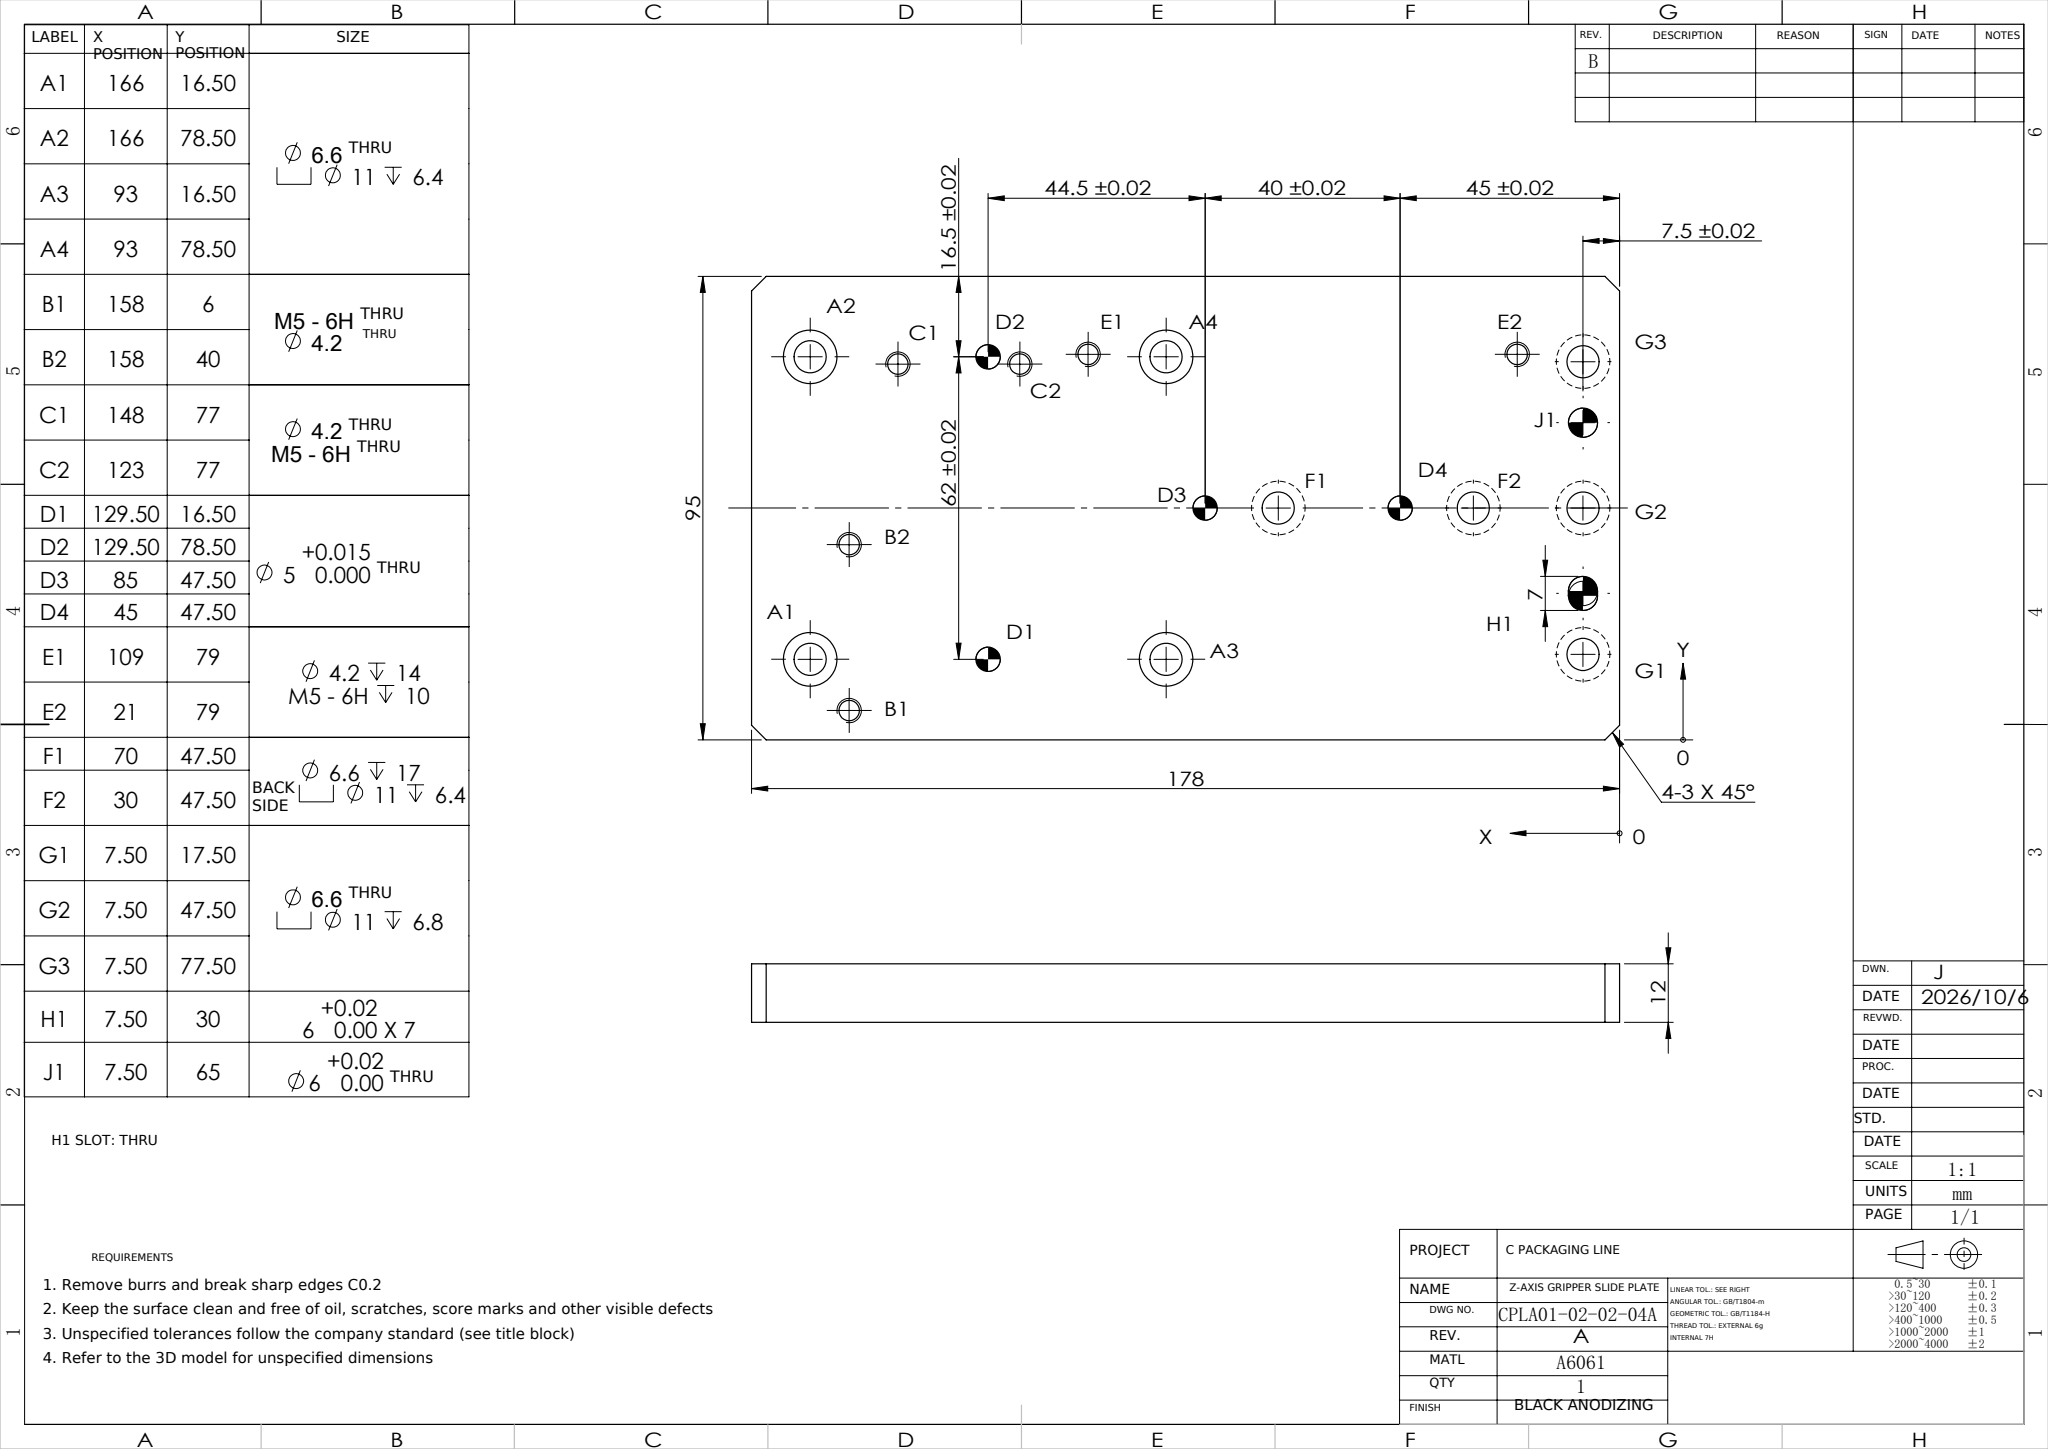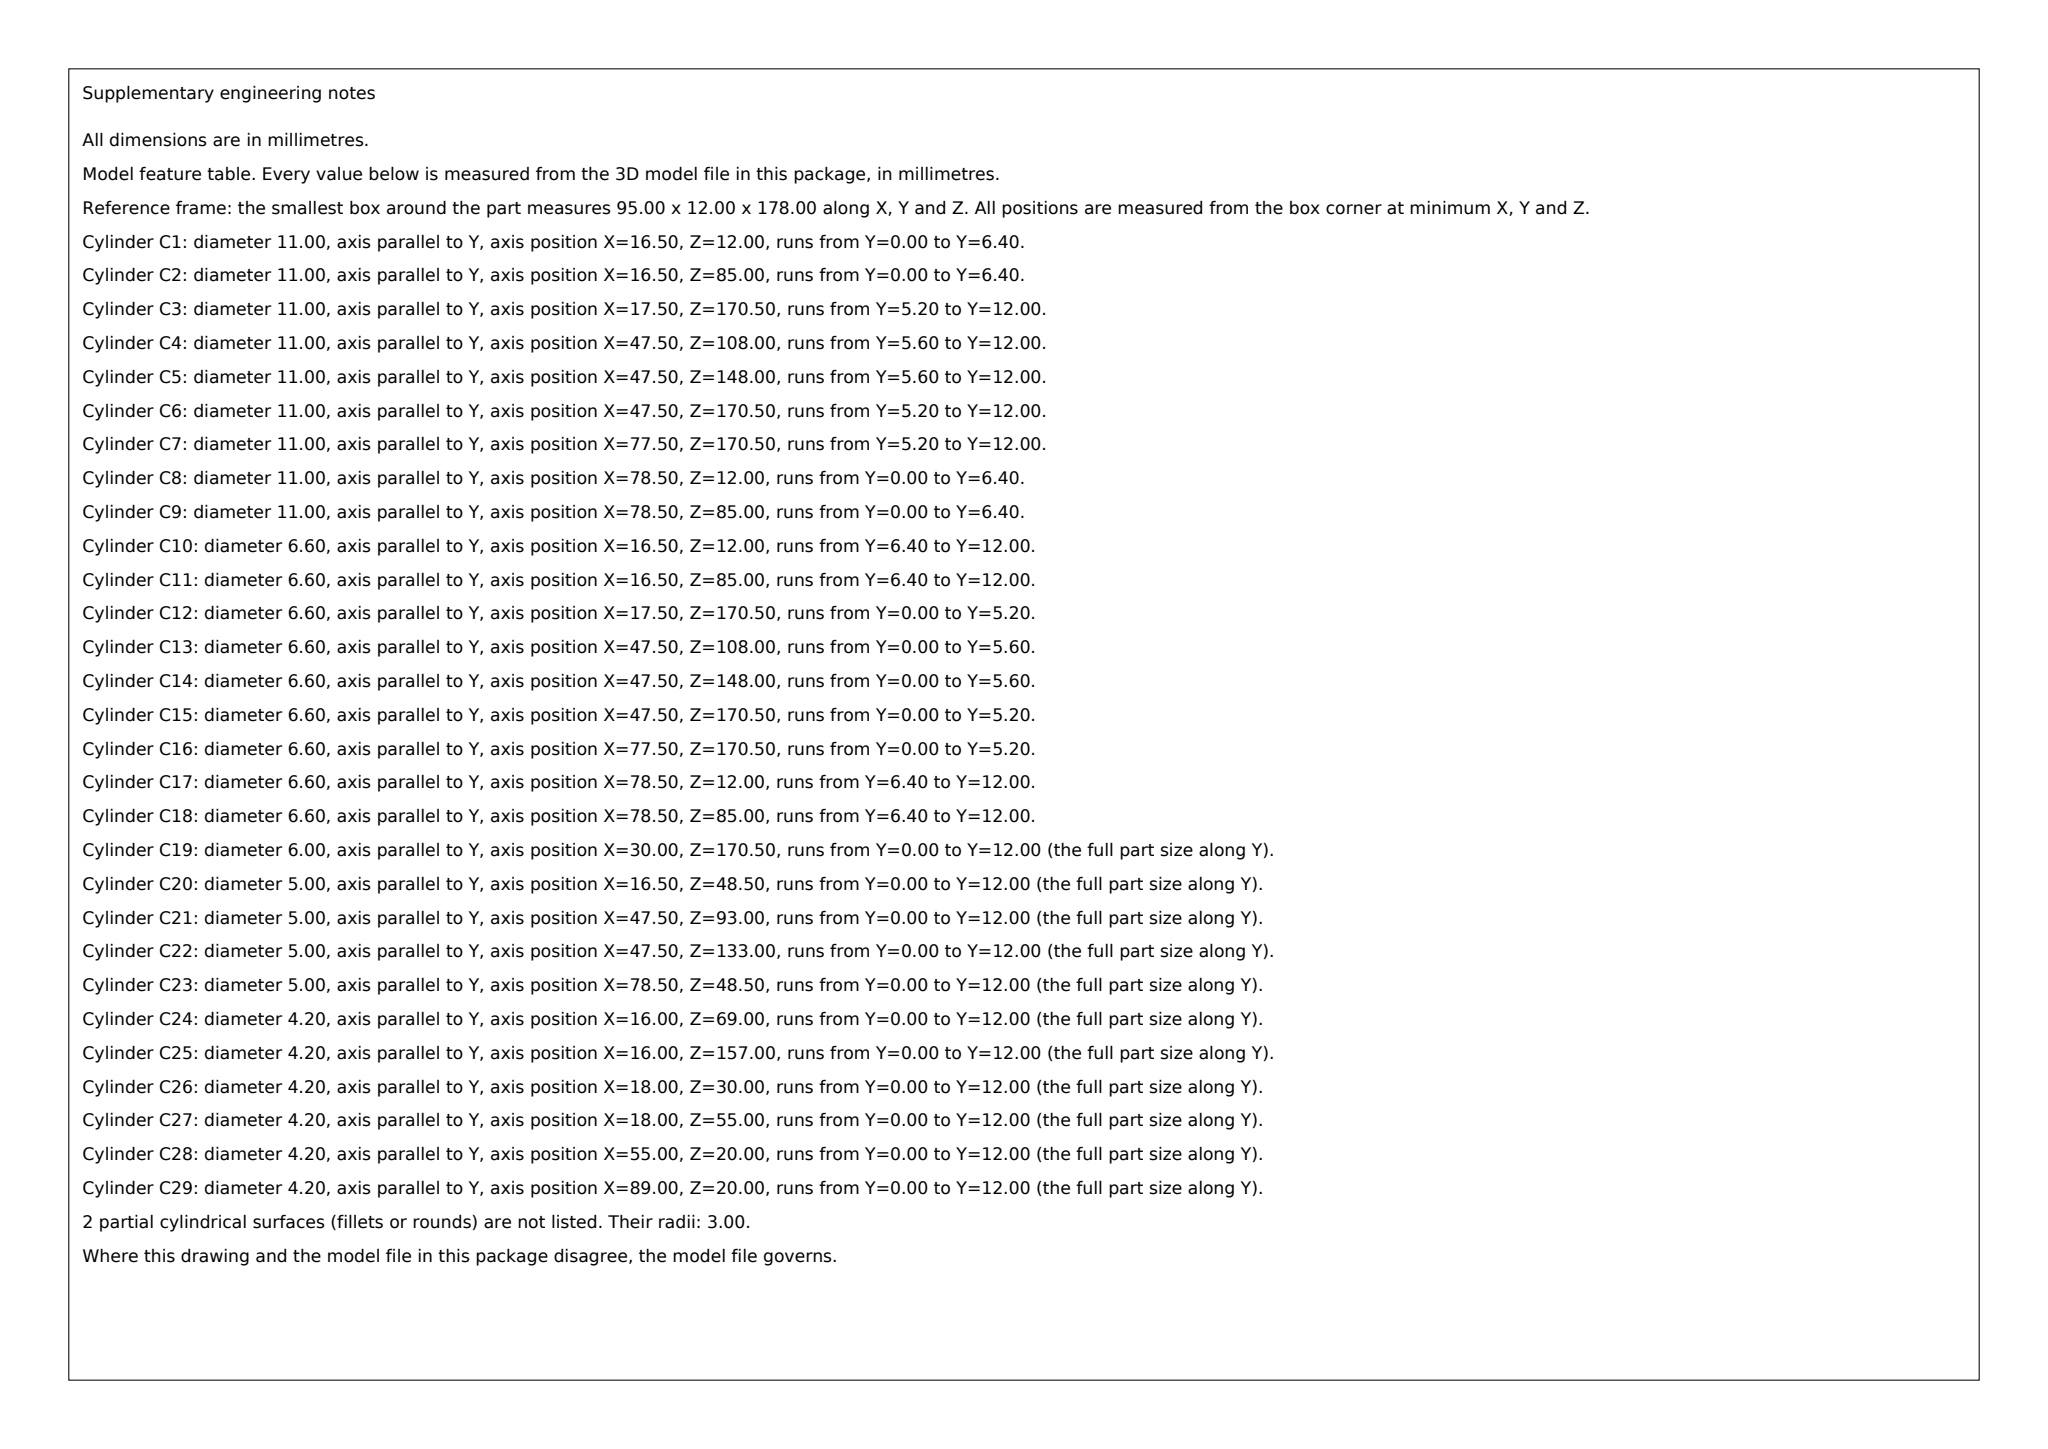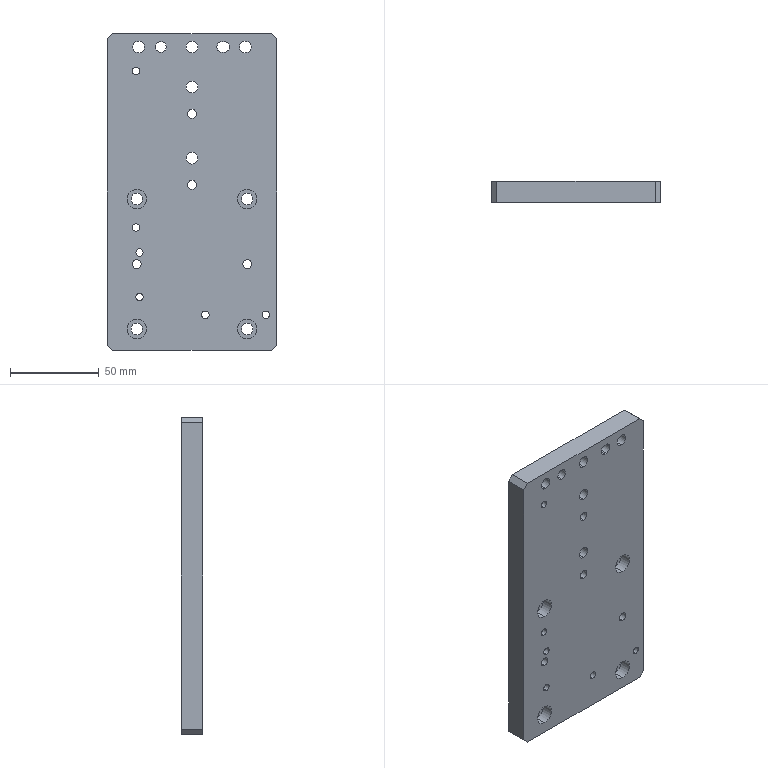Part | SolidWorks | mm | 1 solid | 81 faces | box 95 x 12 x 178 mm | volume 192742 mm3 | cylinder 60 | plane 21 | commonest cylinder face diameters 11 x18 6.6 x18 4.2 x12 5 x8 6 x4
build123d program:
from build123d import *

# Parameters (mm, degrees)
SKETCH1_W                                         = 95
SKETCH1_H                                         = 178
BOSS_EXTRUDE1_DEPTH                               = 12
M6_HEX_SOCKET_HEAD_CAP_SCREW_CBORE2_D             = 6.6
M6_HEX_SOCKET_HEAD_CAP_SCREW_CBORE2_CBORE_D       = 11
M6_HEX_SOCKET_HEAD_CAP_SCREW_CBORE2_CBORE_DEPTH   = 6.4
M6_HEX_SOCKET_HEAD_CAP_SCREW_CBORE1_D             = 6.6
M6_HEX_SOCKET_HEAD_CAP_SCREW_CBORE1_DEPTH         = 17
M6_HEX_SOCKET_HEAD_CAP_SCREW_CBORE1_CBORE_D       = 11
M6_HEX_SOCKET_HEAD_CAP_SCREW_CBORE1_CBORE_DEPTH   = 6.4
M6_HEX_SOCKET_HEAD_CAP_SCREW_CBORE1_TIP           = 1.983
M5_TAPPED_HOLE1_D                                 = 4.2
M5_TAPPED_HOLE1_DEPTH                             = 14
M5_TAPPED_HOLE1_TIP                               = 1.262
CHAMFER1_SIZE                                     = 3
M5_TAPPED_HOLE3_D                                 = 4.2
M5_TAPPED_HOLE4_D                                 = 4.2
F_5_0MM_DOWEL_PIN_HOLE1_D                         = 5
F_5_0MM_DOWEL_PIN_HOLE3_D                         = 5
M6_HEX_SOCKET_HEAD_CAP_SCREW_CBORE1_2_D           = 6.6
M6_HEX_SOCKET_HEAD_CAP_SCREW_CBORE1_2_CBORE_D     = 11
M6_HEX_SOCKET_HEAD_CAP_SCREW_CBORE1_2_CBORE_DEPTH = 6.8
SKETCH24_R                                        = 3
CUT_EXTRUDE1_DEPTH                                = 102.594


with BuildPart() as part:
    # Sketch1 → Boss-Extrude1 (new body)
    with BuildSketch(Plane(origin=(0, 0, 0), x_dir=(1, 0, 0), z_dir=(0, 1, 0))):
        Rectangle(SKETCH1_W, SKETCH1_H)
    extrude(amount=BOSS_EXTRUDE1_DEPTH)

    # M6 Hex Socket Head Cap Screw CBORE2 (through all)
    with Locations(Plane(origin=(0, 0, 0), x_dir=(-1, 0, 0), z_dir=(0, -1, 0))):
        with Locations((-31, 77), (-31, 4), (31, 77), (31, 4)):
            CounterBoreHole(M6_HEX_SOCKET_HEAD_CAP_SCREW_CBORE2_D / 2, M6_HEX_SOCKET_HEAD_CAP_SCREW_CBORE2_CBORE_D / 2, M6_HEX_SOCKET_HEAD_CAP_SCREW_CBORE2_CBORE_DEPTH)

    # M6 Hex Socket Head Cap Screw CBORE1
    with Locations(Plane(origin=(0, 12, 0), x_dir=(1, 0, 0), z_dir=(0, 1, 0))):
        with Locations((0, -59), (0, -19)):
            CounterBoreHole(M6_HEX_SOCKET_HEAD_CAP_SCREW_CBORE1_D / 2, M6_HEX_SOCKET_HEAD_CAP_SCREW_CBORE1_CBORE_D / 2, M6_HEX_SOCKET_HEAD_CAP_SCREW_CBORE1_CBORE_DEPTH, depth=M6_HEX_SOCKET_HEAD_CAP_SCREW_CBORE1_DEPTH)
            with Locations((0, 0, -(M6_HEX_SOCKET_HEAD_CAP_SCREW_CBORE1_DEPTH + M6_HEX_SOCKET_HEAD_CAP_SCREW_CBORE1_TIP / 2))):  # 118° drill point
                Cone(0, M6_HEX_SOCKET_HEAD_CAP_SCREW_CBORE1_D / 2, M6_HEX_SOCKET_HEAD_CAP_SCREW_CBORE1_TIP, mode=Mode.SUBTRACT)

    # M5 Tapped Hole1
    with Locations(Plane(origin=(0, 0, 0), x_dir=(-1, 0, 0), z_dir=(0, -1, 0))):
        with Locations((31.5, -68), (31.5, 20)):
            Hole(M5_TAPPED_HOLE1_D / 2, depth=M5_TAPPED_HOLE1_DEPTH)
            with Locations((0, 0, -(M5_TAPPED_HOLE1_DEPTH + M5_TAPPED_HOLE1_TIP / 2))):  # 118° drill point
                Cone(0, M5_TAPPED_HOLE1_D / 2, M5_TAPPED_HOLE1_TIP, mode=Mode.SUBTRACT)

    # Chamfer1
    chamfer1_edges = [part.edges().sort_by_distance(p)[0] for p in [
        (-47.5, 6, -89),
        (47.5, 6, -89),
        (47.5, 6, 89),
        (-47.5, 6, 89),
    ]]
    chamfer(chamfer1_edges, length=CHAMFER1_SIZE)

    # M5 Tapped Hole3 (through all)
    with Locations(Plane(origin=(0, 0, 0), x_dir=(-1, 0, 0), z_dir=(0, -1, 0))):
        with Locations((29.5, 59), (29.5, 34)):
            Hole(M5_TAPPED_HOLE3_D / 2)

    # M5 Tapped Hole4 (through all)
    with Locations(Plane(origin=(0, 0, 0), x_dir=(-1, 0, 0), z_dir=(0, -1, 0))):
        with Locations((-41.5, 69), (-7.5, 69)):
            Hole(M5_TAPPED_HOLE4_D / 2)

    # 5.0mm Dowel Pin Hole1 (through all)
    with Locations(Plane(origin=(0, 0, 0), x_dir=(-1, 0, 0), z_dir=(0, -1, 0))):
        with Locations((-31, 40.5), (31, 40.5)):
            Hole(F_5_0MM_DOWEL_PIN_HOLE1_D / 2)

    # 5.0mm Dowel Pin Hole3 (through all)
    with Locations(Plane(origin=(0, 12, 0), x_dir=(1, 0, 0), z_dir=(0, 1, 0))):
        with Locations((0, -44), (0, -4)):
            Hole(F_5_0MM_DOWEL_PIN_HOLE3_D / 2)

    # M6 Hex Socket Head Cap Screw CBORE1_2 (through all)
    with Locations(Plane(origin=(0, 12, 0), x_dir=(1, 0, 0), z_dir=(0, 1, 0))):
        with Locations((30, -81.5), (-30, -81.5), (0, -81.5)):
            CounterBoreHole(M6_HEX_SOCKET_HEAD_CAP_SCREW_CBORE1_2_D / 2, M6_HEX_SOCKET_HEAD_CAP_SCREW_CBORE1_2_CBORE_D / 2, M6_HEX_SOCKET_HEAD_CAP_SCREW_CBORE1_2_CBORE_DEPTH)

    # Sketch24 → Cut-Extrude1 (cut, through all)
    with BuildSketch(Plane(origin=(0, 12, 0), x_dir=(1, 0, 0), z_dir=(0, 1, 0))):
        with Locations(Location((-17.5, -81.5, 0), (0, 0, 270))):
            Circle(SKETCH24_R)
        with BuildLine():
            Line((17, -78.5), (18, -78.5))
            ThreePointArc((18, -78.5), (21, -81.5), (18, -84.5))
            Line((18, -84.5), (17, -84.5))
            ThreePointArc((17, -84.5), (14, -81.5), (17, -78.5))
        make_face()
    extrude(amount=-CUT_EXTRUDE1_DEPTH, mode=Mode.SUBTRACT)


solid = part.part